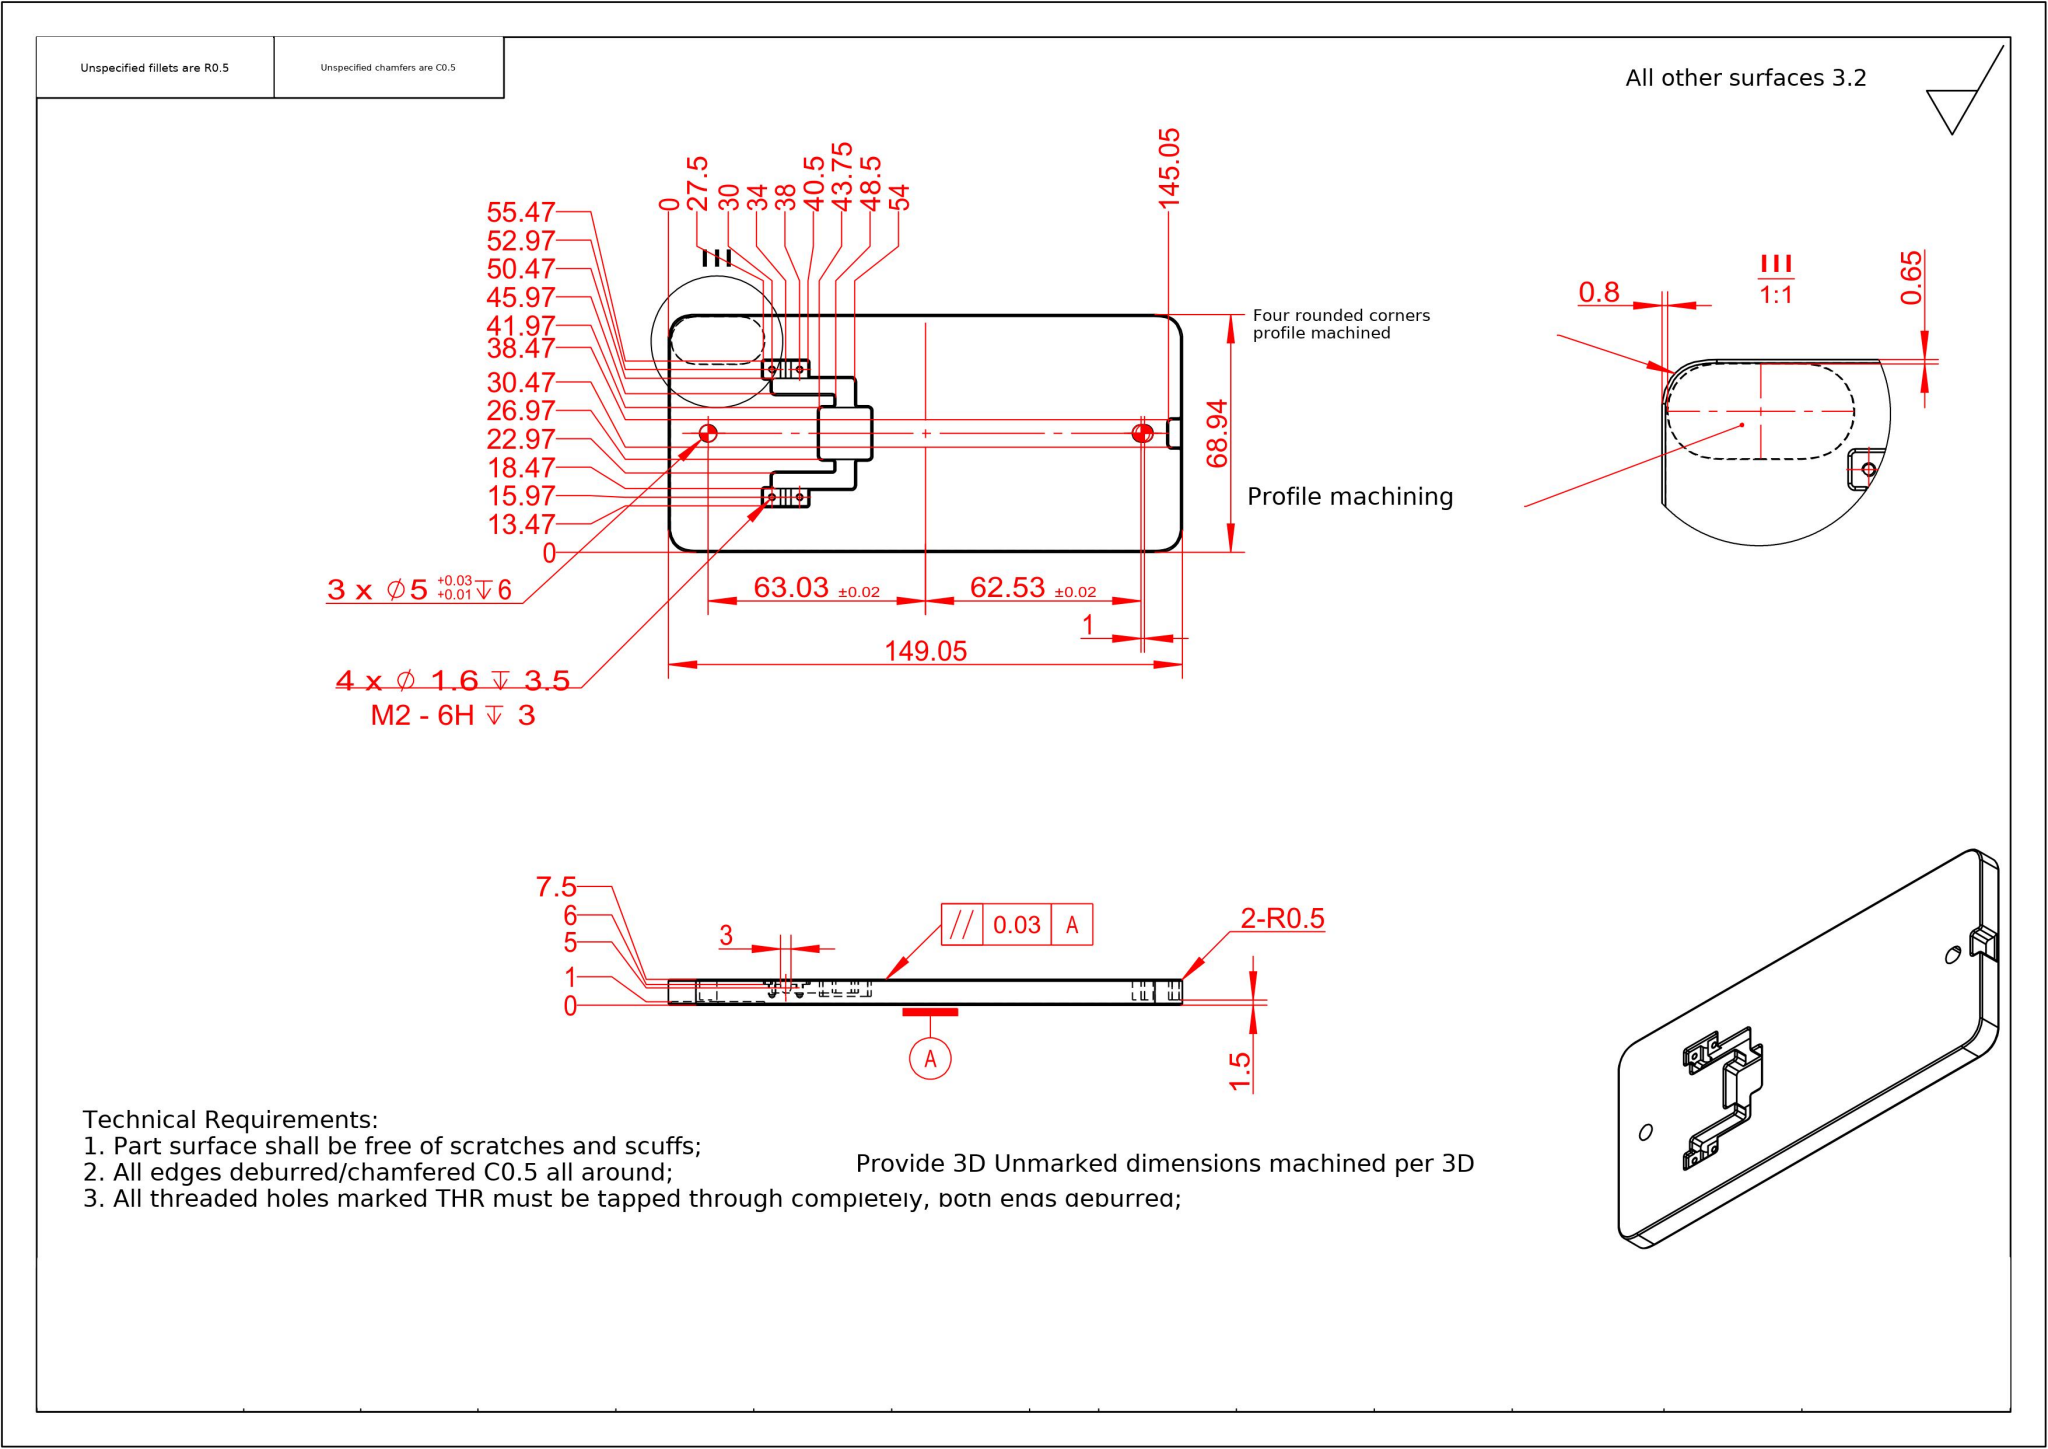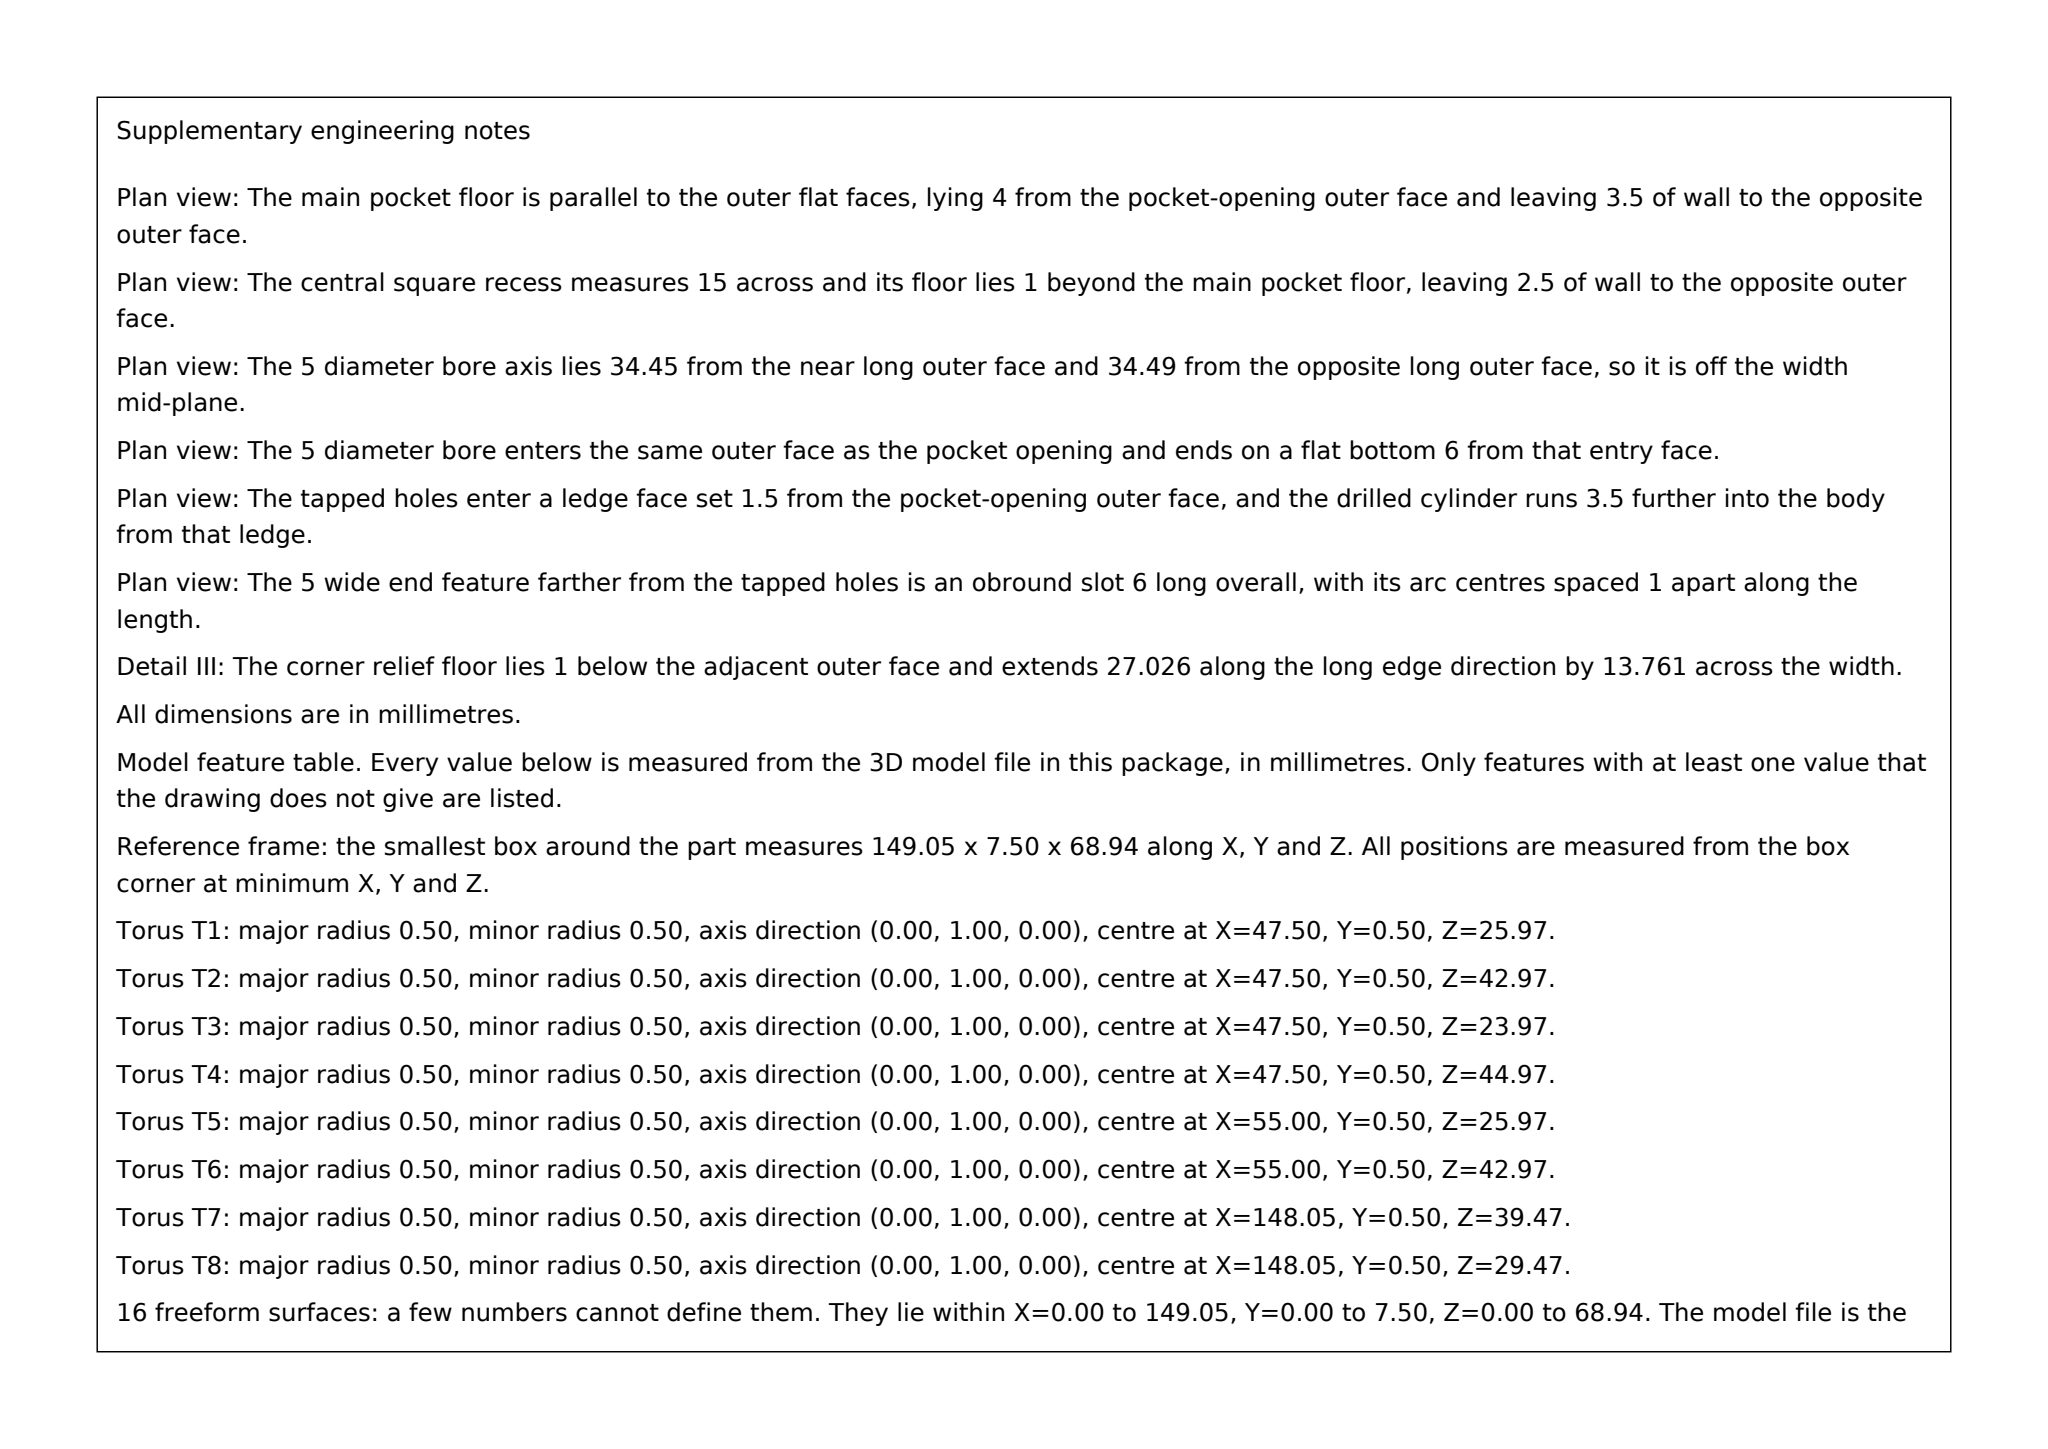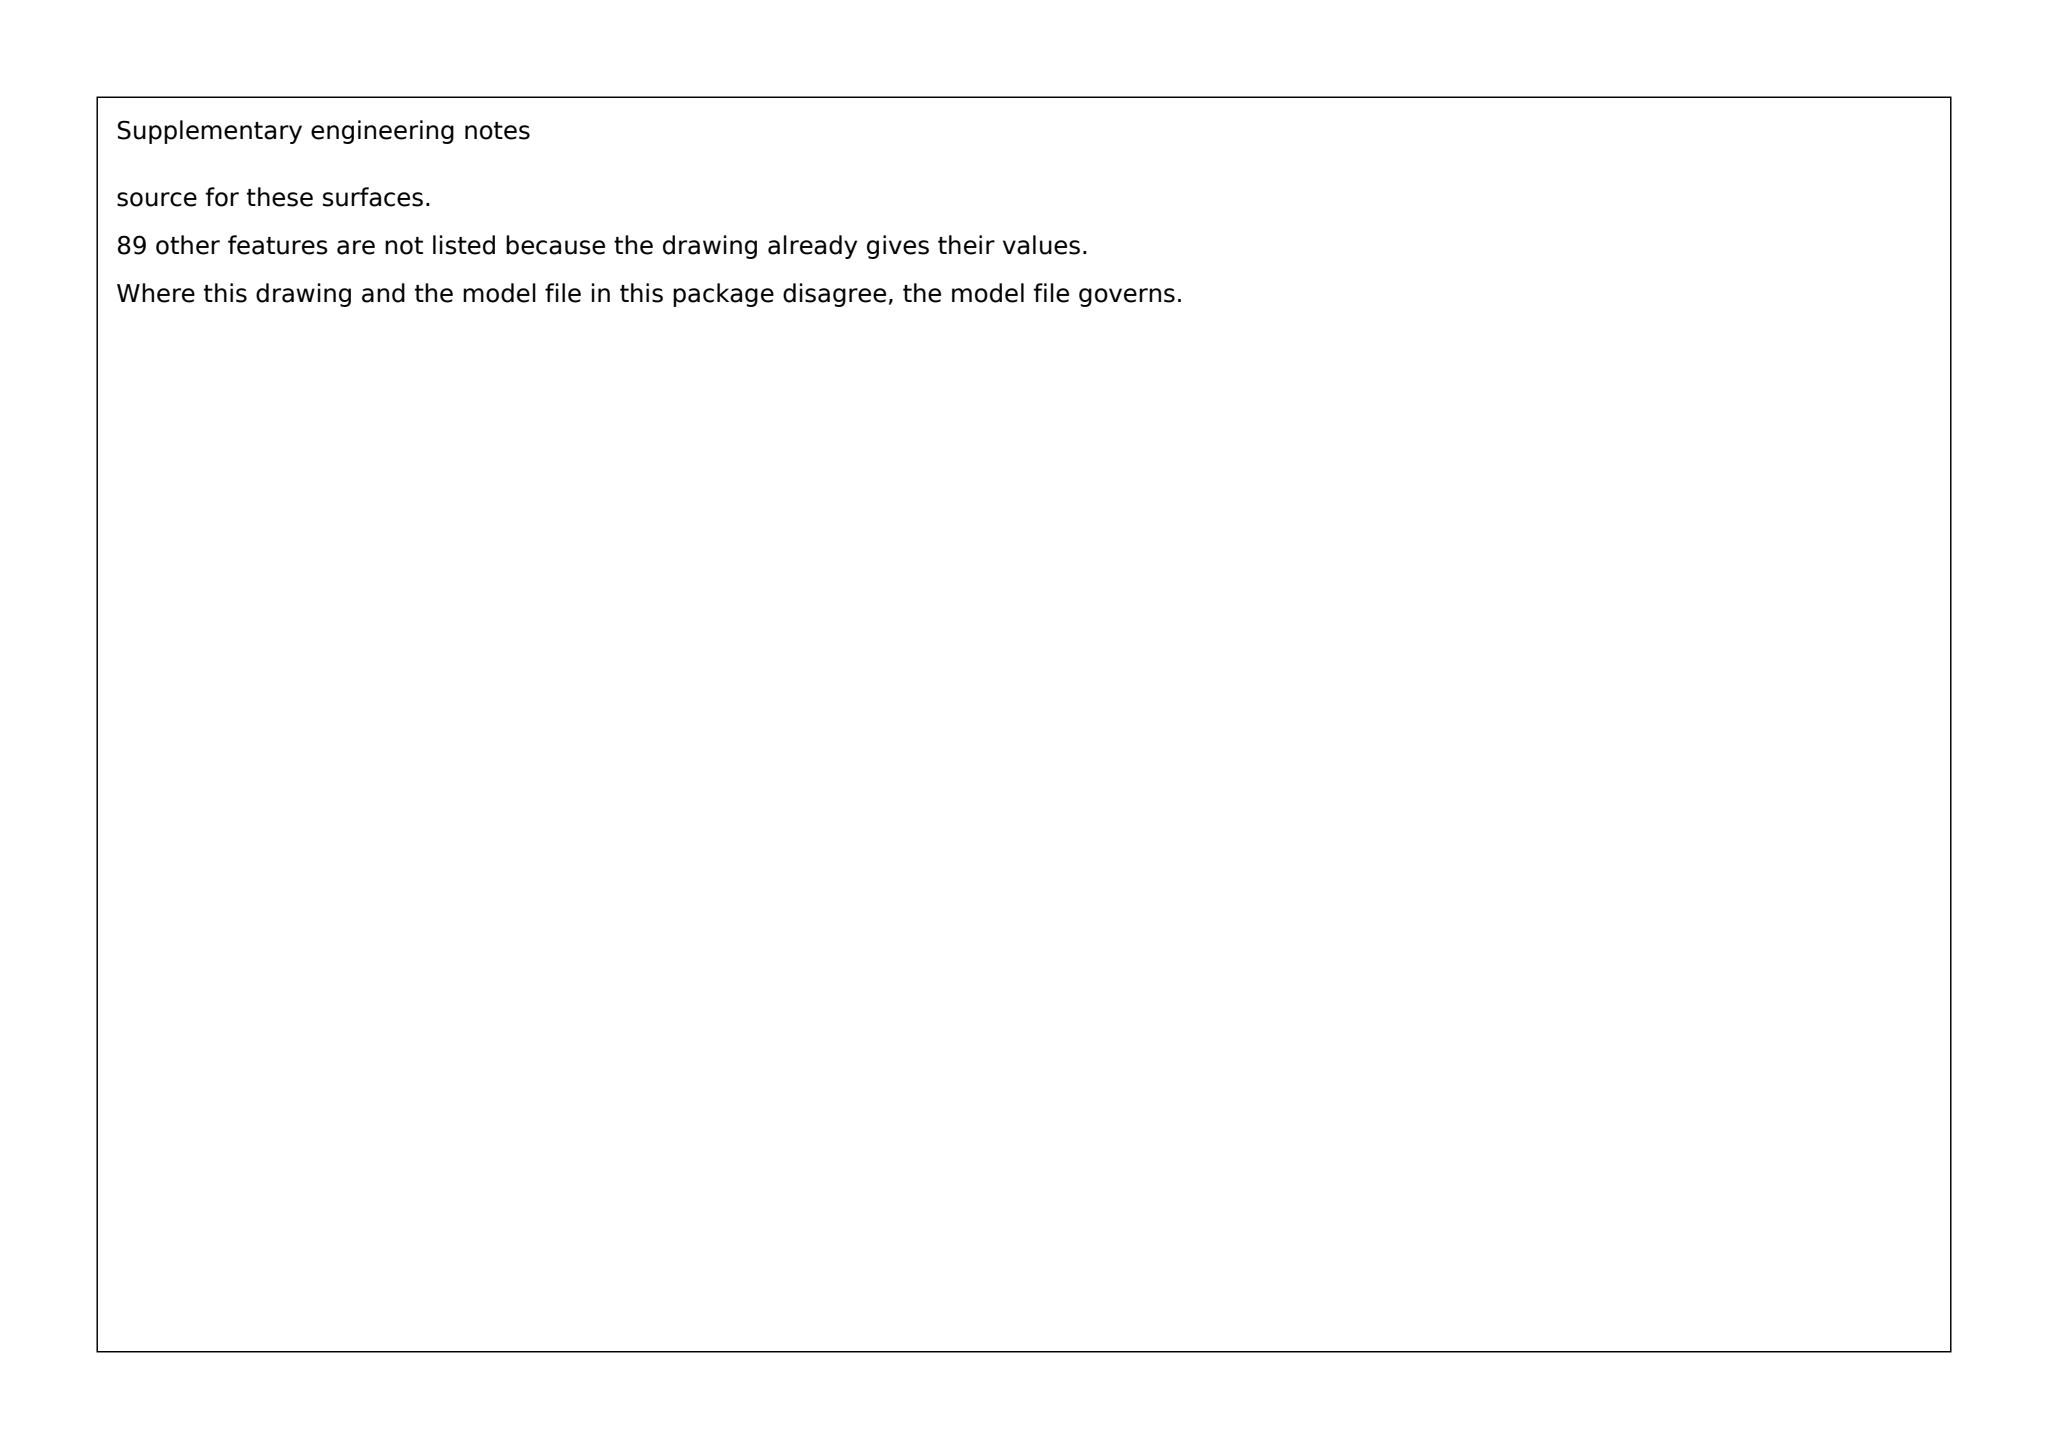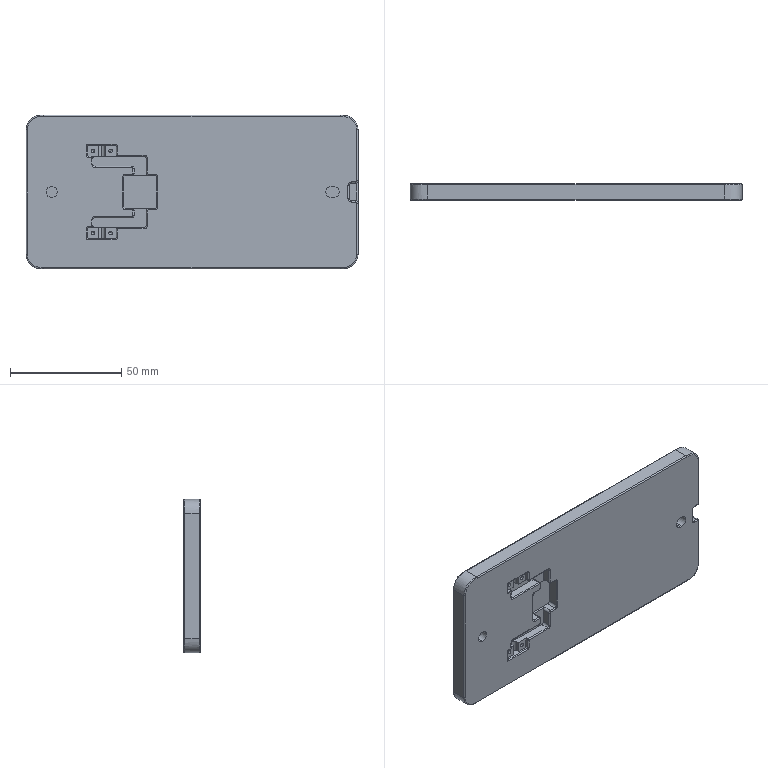Part | SolidWorks | mm | 1 solid | 187 faces | box 149.05 x 7.5 x 68.94 mm | volume 73473 mm3 | cylinder 83 | plane 50 | torus 26 | spline 16 | cone 8 | sphere 4 | commonest cylinder face diameters 1 x47 2 x20 1.6 x8 5 x4 3 x4
Drawing notes:
3RD Ø5 +0.03/+0.01 DP 6 AT X138.05, Z34.49 (ON HORIZ CL) | from the solid: Ø5 y-axis cyls at x=11.51, 137.06, 138.06, all z=34.49, len 6; datum x=0.01, z=0
STEPPED POCKET INT CNRS: 4X Ø3 (R1.5) DP 5 AT X34.0, Y2.5 | from the solid: cylinders [3.0,'z',[34.01,2.5,null],5.0,count 4]
RH TAB: X145.05 TO 149.05, 10 WIDE (Z29.47-39.47), ON HORIZ CL | from the solid: x planes 145.06 & 149.06; z-axis fillet at x=148.56,y=6.5 len 10; tab holes z 29.47/39.47
RH TAB: 2X Ø2 DP 5.5 AT X146.05, Z31.47 & Z37.47 | from the solid: [2.0,'y',[146.06,null,31.47],3.5... len 5.5] and [2.0,'y',[146.06,null,37.47],5.5]
RH TAB: 2X Ø2 DP 6 AT X148.05, Z29.47 & Z39.47 | from the solid: [2.0,'y',[148.06,null,29.47],6.0] and [2.0,'y',[148.06,null,39.47],6.0]
CONN CUTOUT INT CORNERS R1 (Ø2): DP 3.5 TYP, DP 4.5 AT X44.76 & X57.76 | from the solid: cylinders dia 2.0 axis y at x=31.01/47.51/53.01/55.01 len 3.5; x=44.76/57.76 len 4.5
R1 CORNER Z: 19.47,21.97,23.97,25.97,27.97, SYM ABT CL Z34.47 | from the solid: dia2 y-axis cyl z=19.47,21.97,23.97,25.97,27.97 mirrored at 49.47,46.97,44.97,42.97,40.97 (sum 68.94)
ADD ORDINATE X32.5 & X35.5: STEPPED POCKET / CONN STEP WALLS | from the solid: axis_planes x=32.51 (2) and x=35.51 (2); ordinate datum = x face 0.01
CTR TAB SLOT 5 WIDE: Z31.99 TO Z36.99, SYM ABT CL Z34.47 | from the solid: axis_planes z=31.99 (1) and z=36.99 (1), 5.0 apart, centred on 34.49 CL of 68.94
ADD SIDE VIEW ORDINATES Y1.5, Y4 & Y6.5 FOR DEPTH STEPS | from the solid: axis_planes y=1.5 (4), y=4.0 (2), y=6.5 (1) not in 0/1/5/6/7.5 chain
4X OUTER PROFILE CORNER R6.4 (vertical corners of 149.05 x 68.94 outline), TANGENT TO BOTH ADJACENT EDGES, FULL 7.5 THICKNESS | from the solid: bbox_xyz Z = 68.94 with dia 1.0 z-axis edge-fillet cylinder at x=0.51 of length 56.14 (68.94 - 2 x 6.4 = 56.14), i.e. straight edge runs Z6.4 to Z62.54, giving R6.4 profile corners